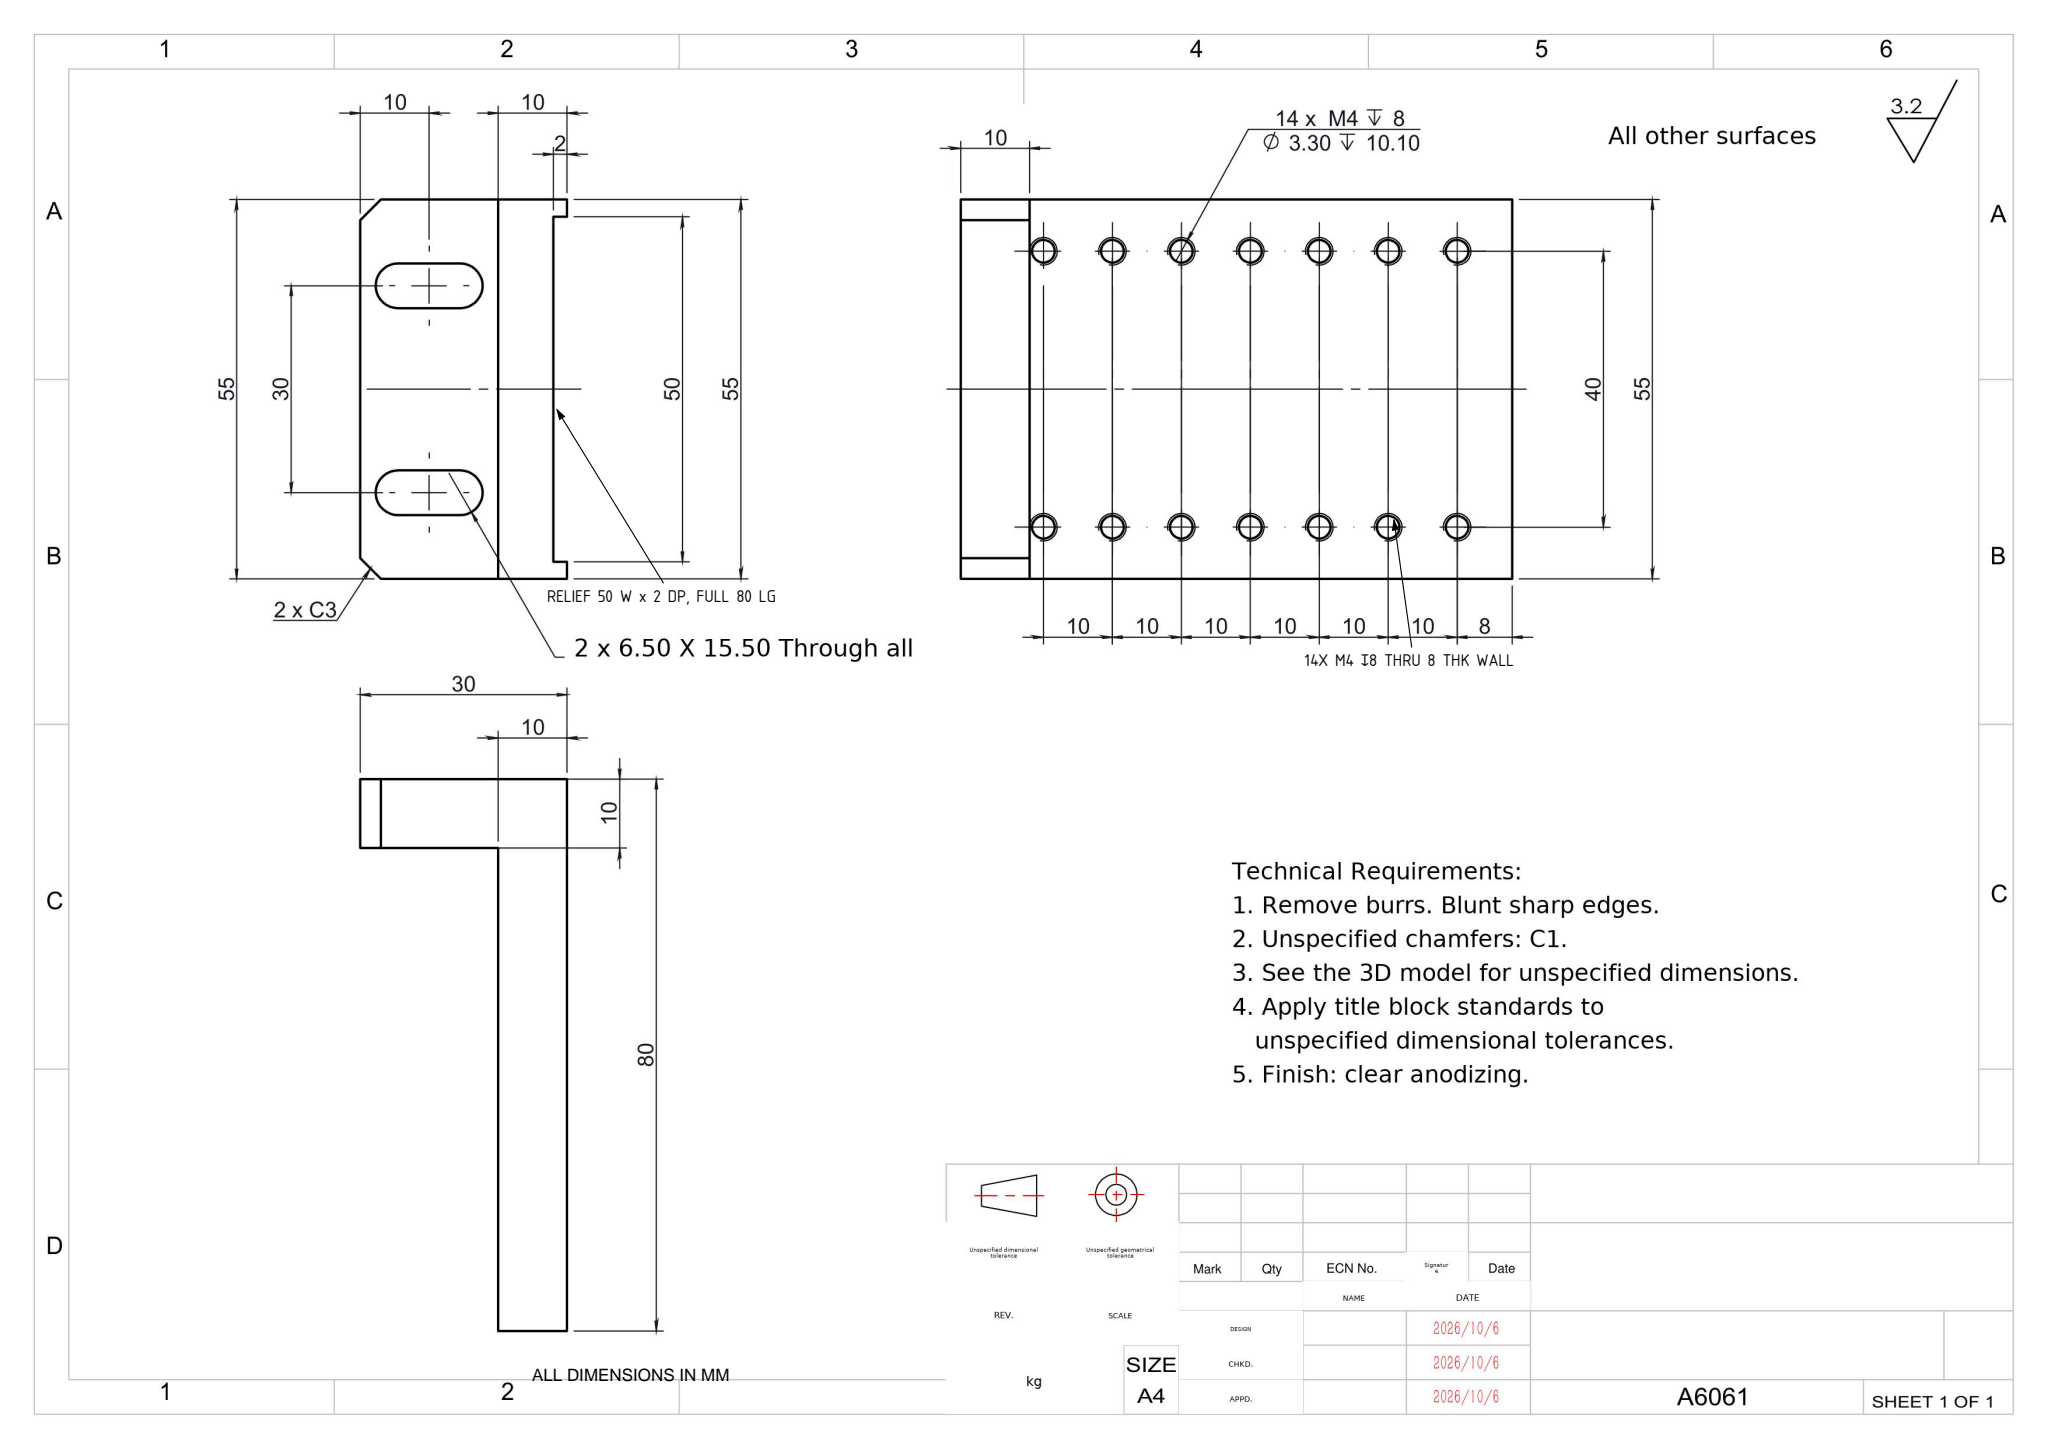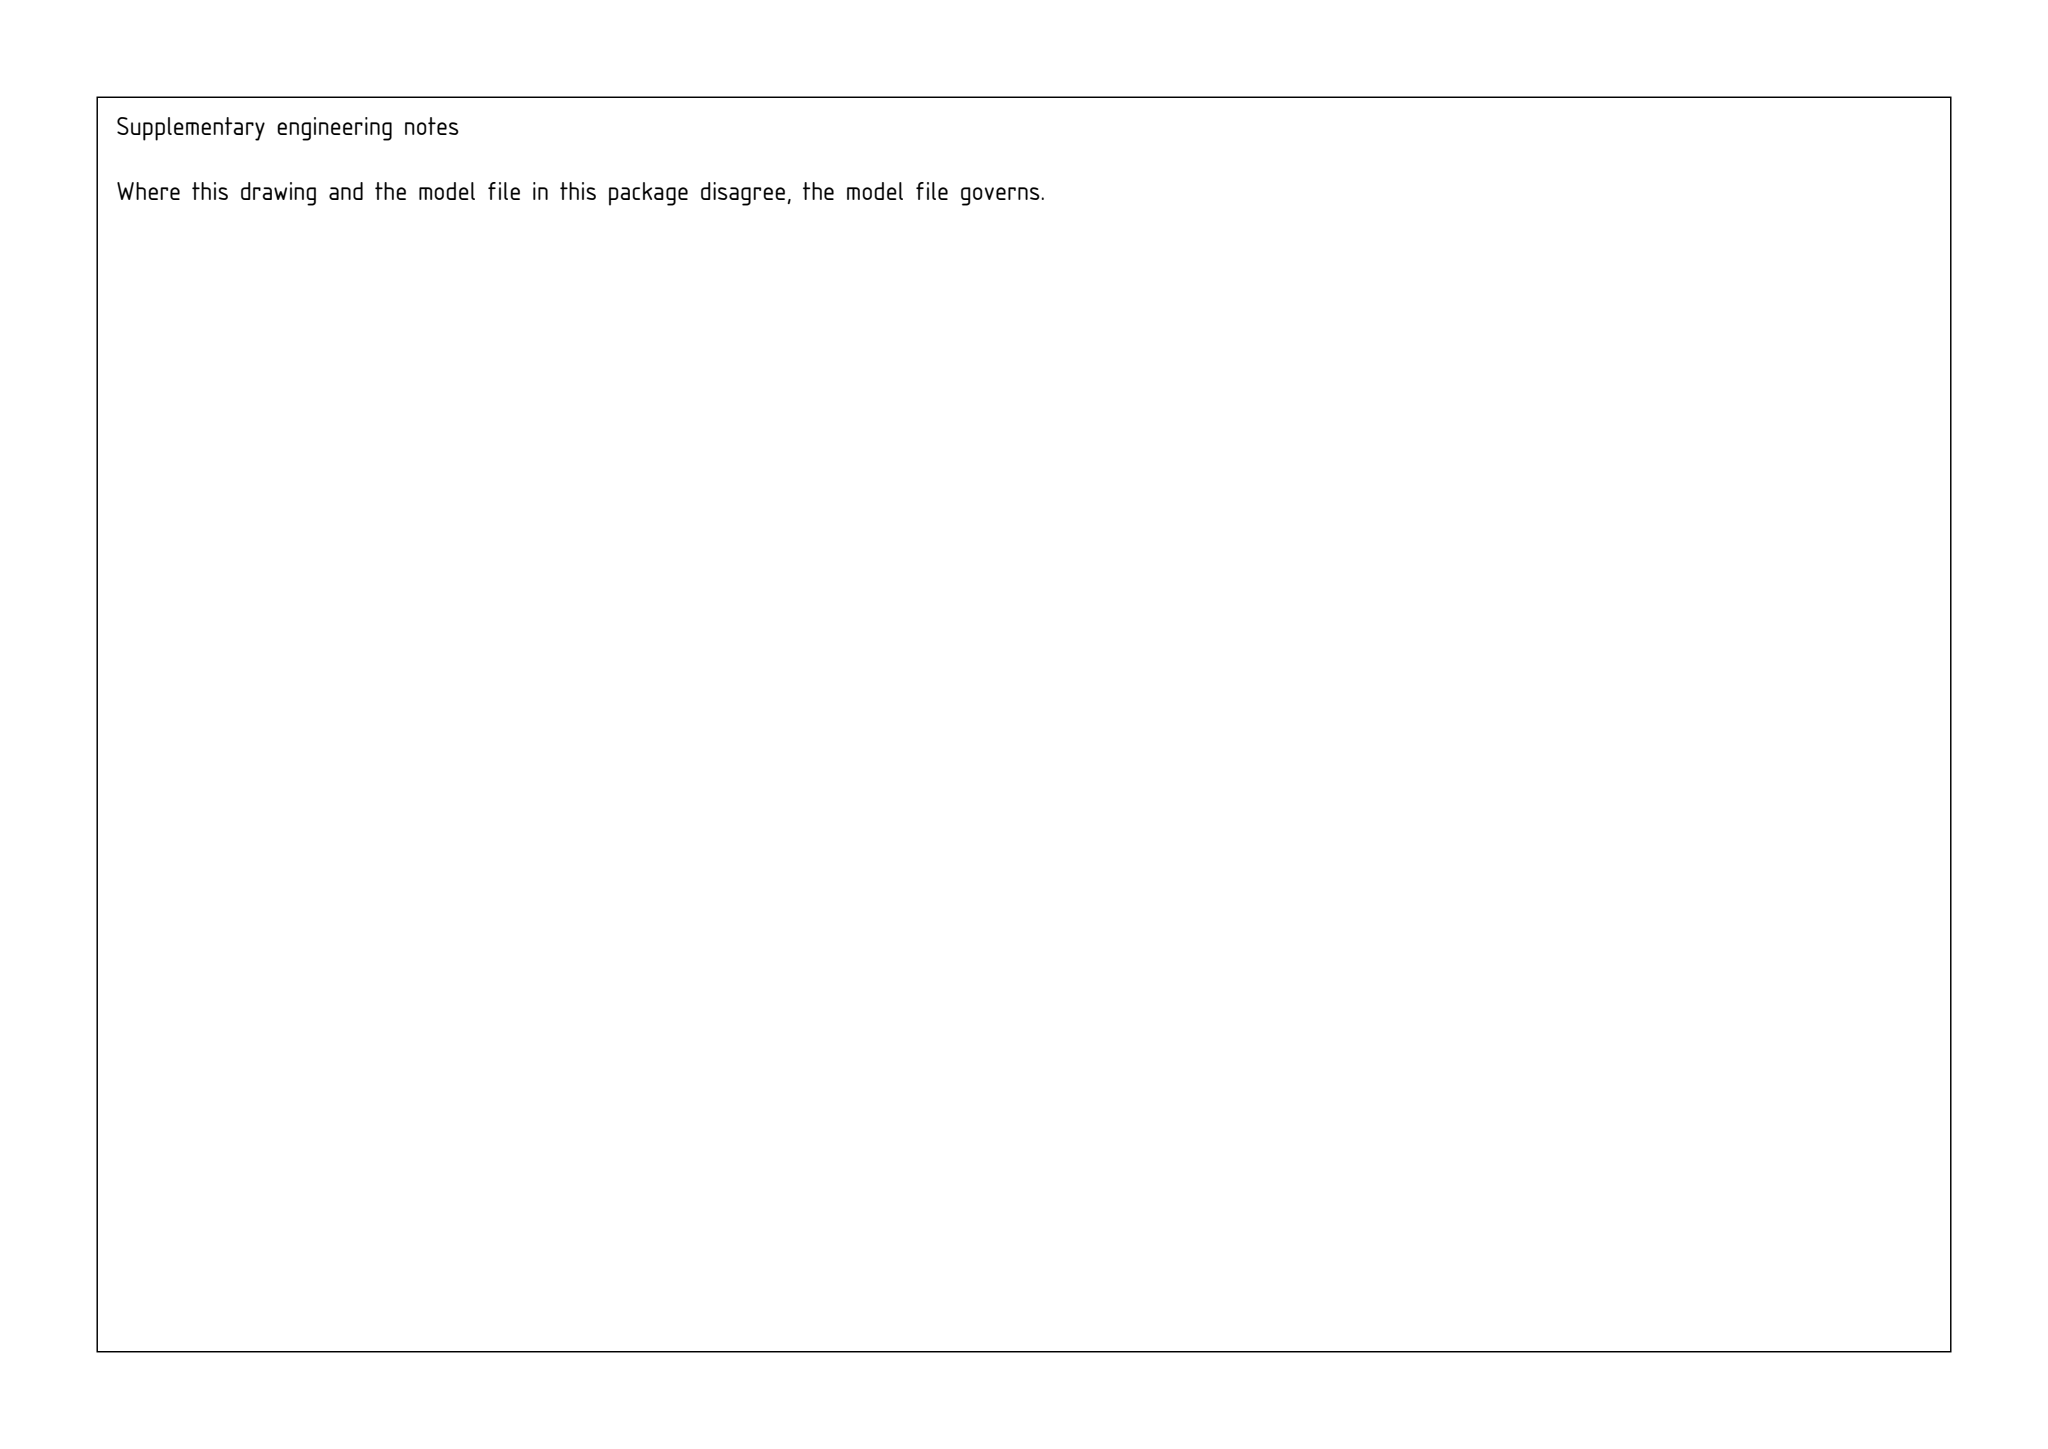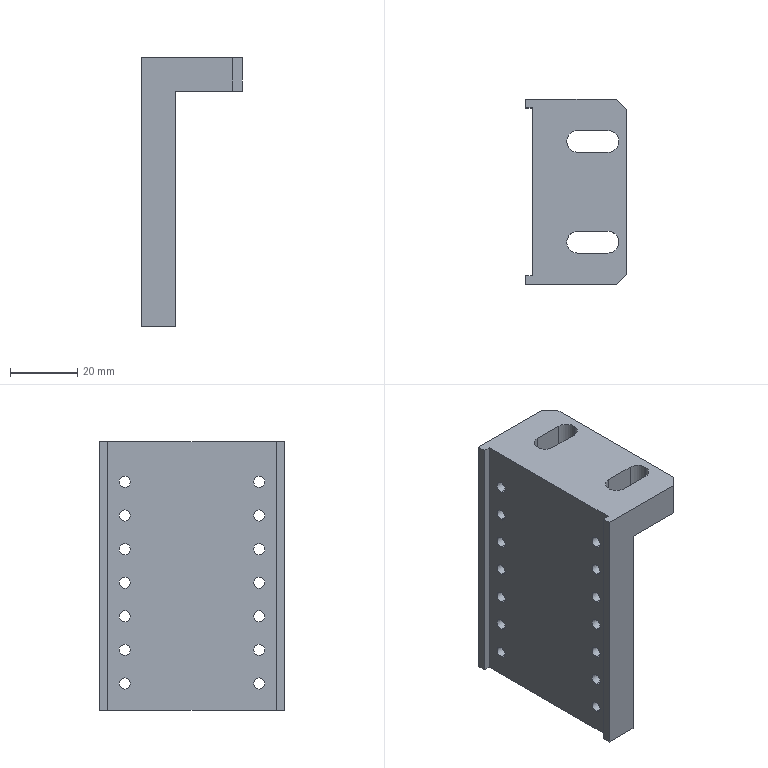Part | SolidWorks | mm | material A6061 | 1 solid | 52 faces | box 30 x 55 x 80 mm | volume 44118 mm3 | cylinder 34 | plane 18 | commonest cylinder face diameters 3.3 x28 6.5 x6
Drawing notes:
REAR RELIEF 50 W x 2 DP RUNS FULL 80 LG, 2.5 FROM EA SIDE | from the solid: x planes 0/2, y planes 2.5/52.5, z 0-80: 2 deep recess full height, 50 wide
14 x M4 HT 8 FROM FRONT FACE; THRU 8 THK WALL INTO REAR RELIEF | from the solid: 14 x Ø3.3 holes, axis x, length 8, spanning x=2 (relief floor) to x=10 front face